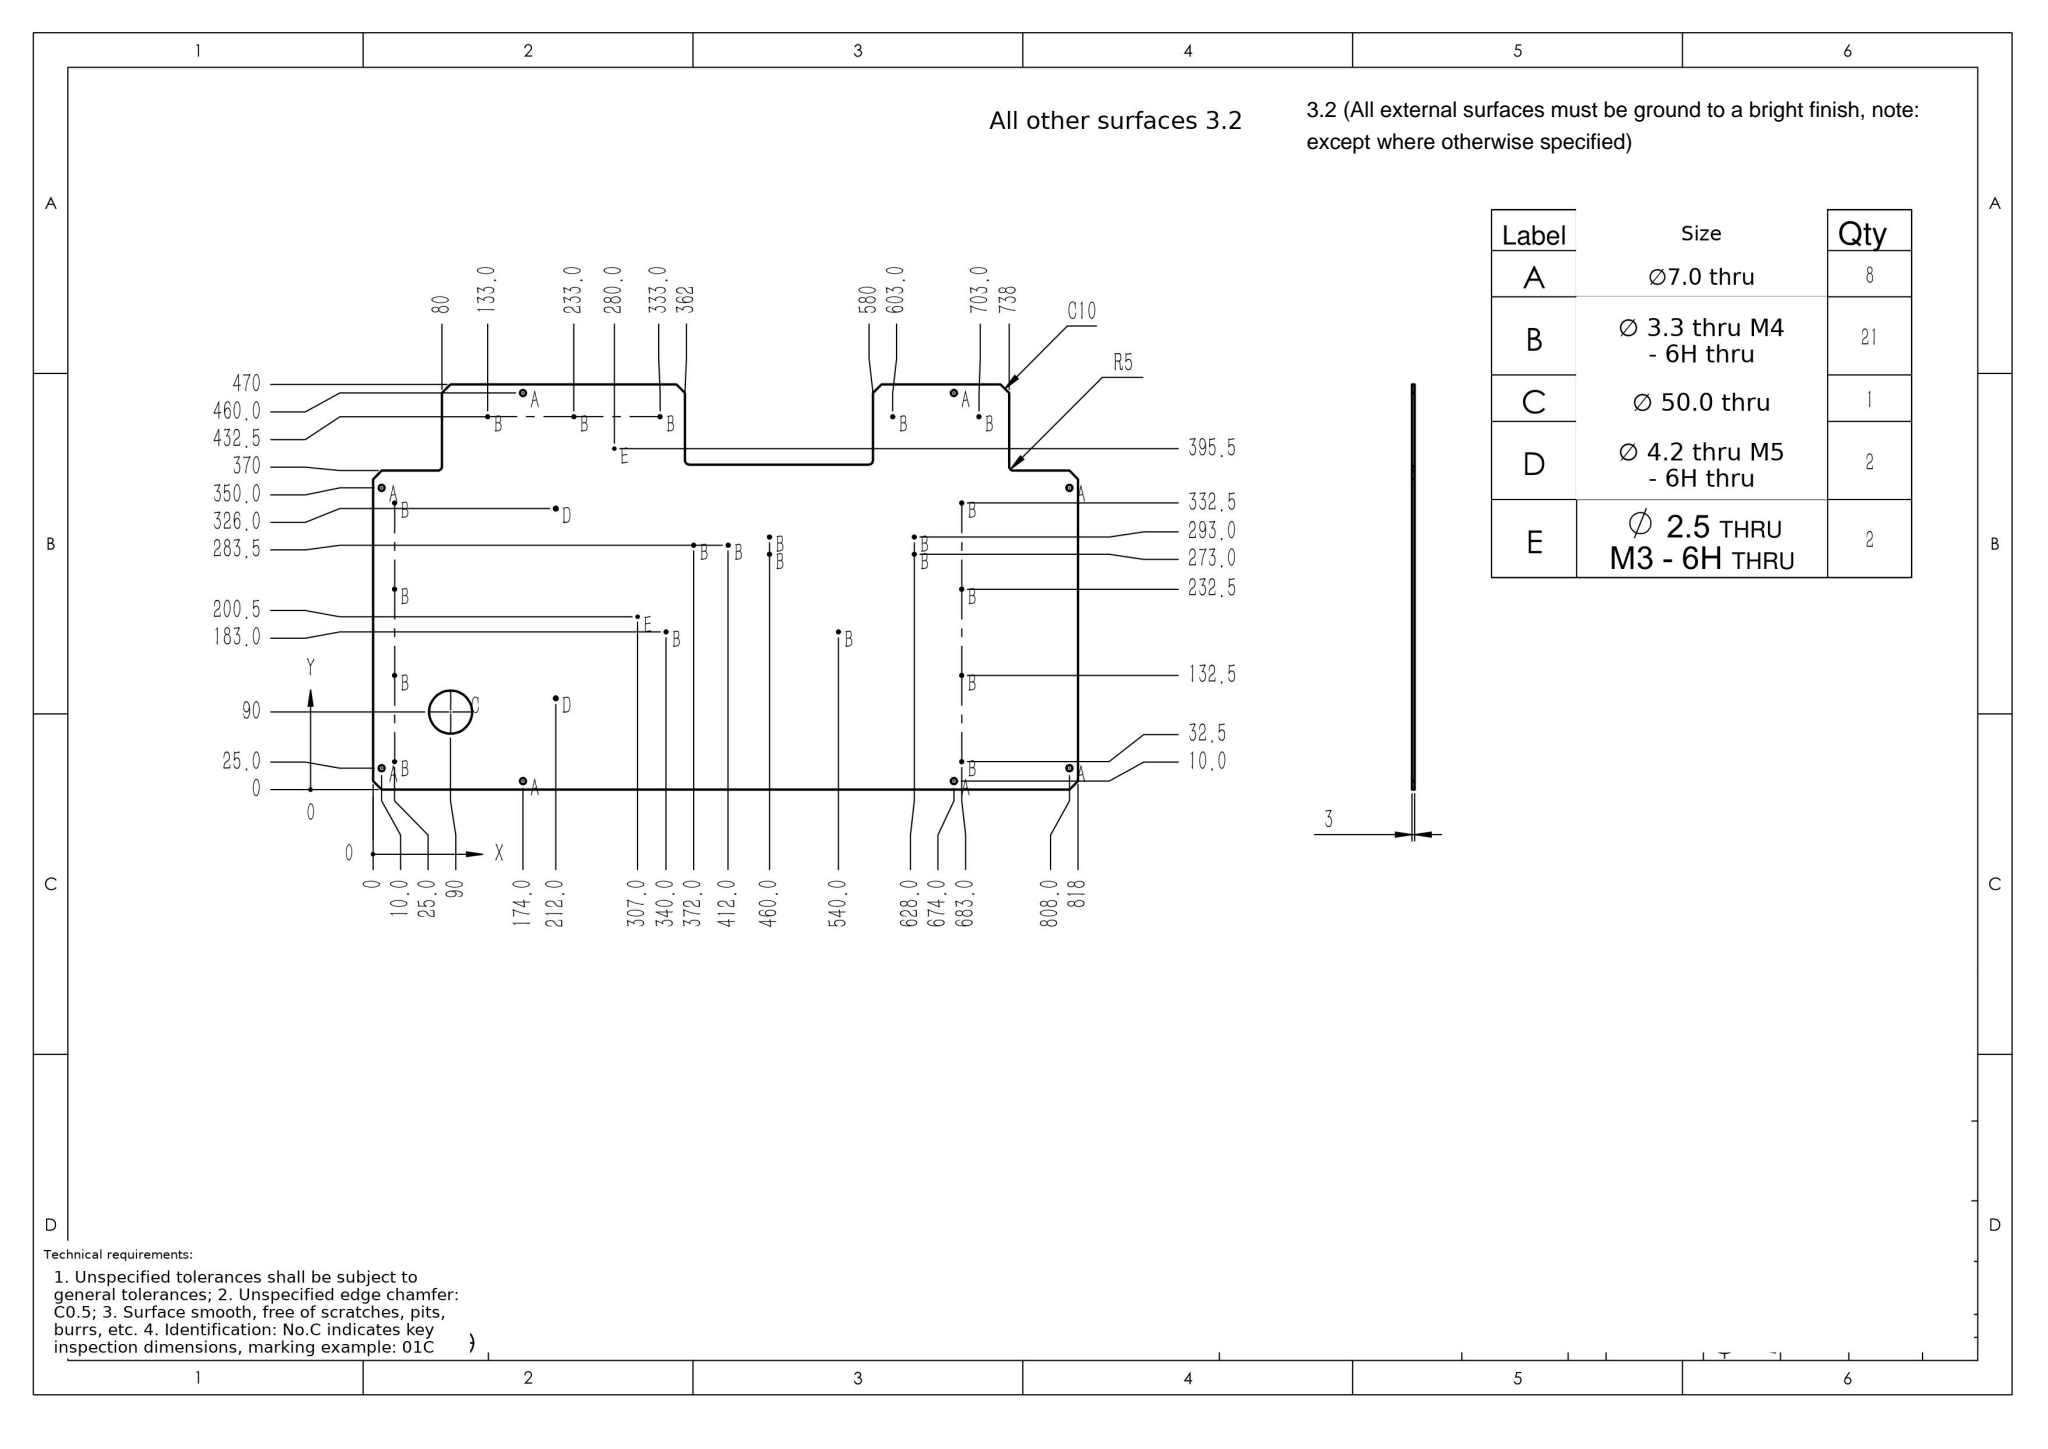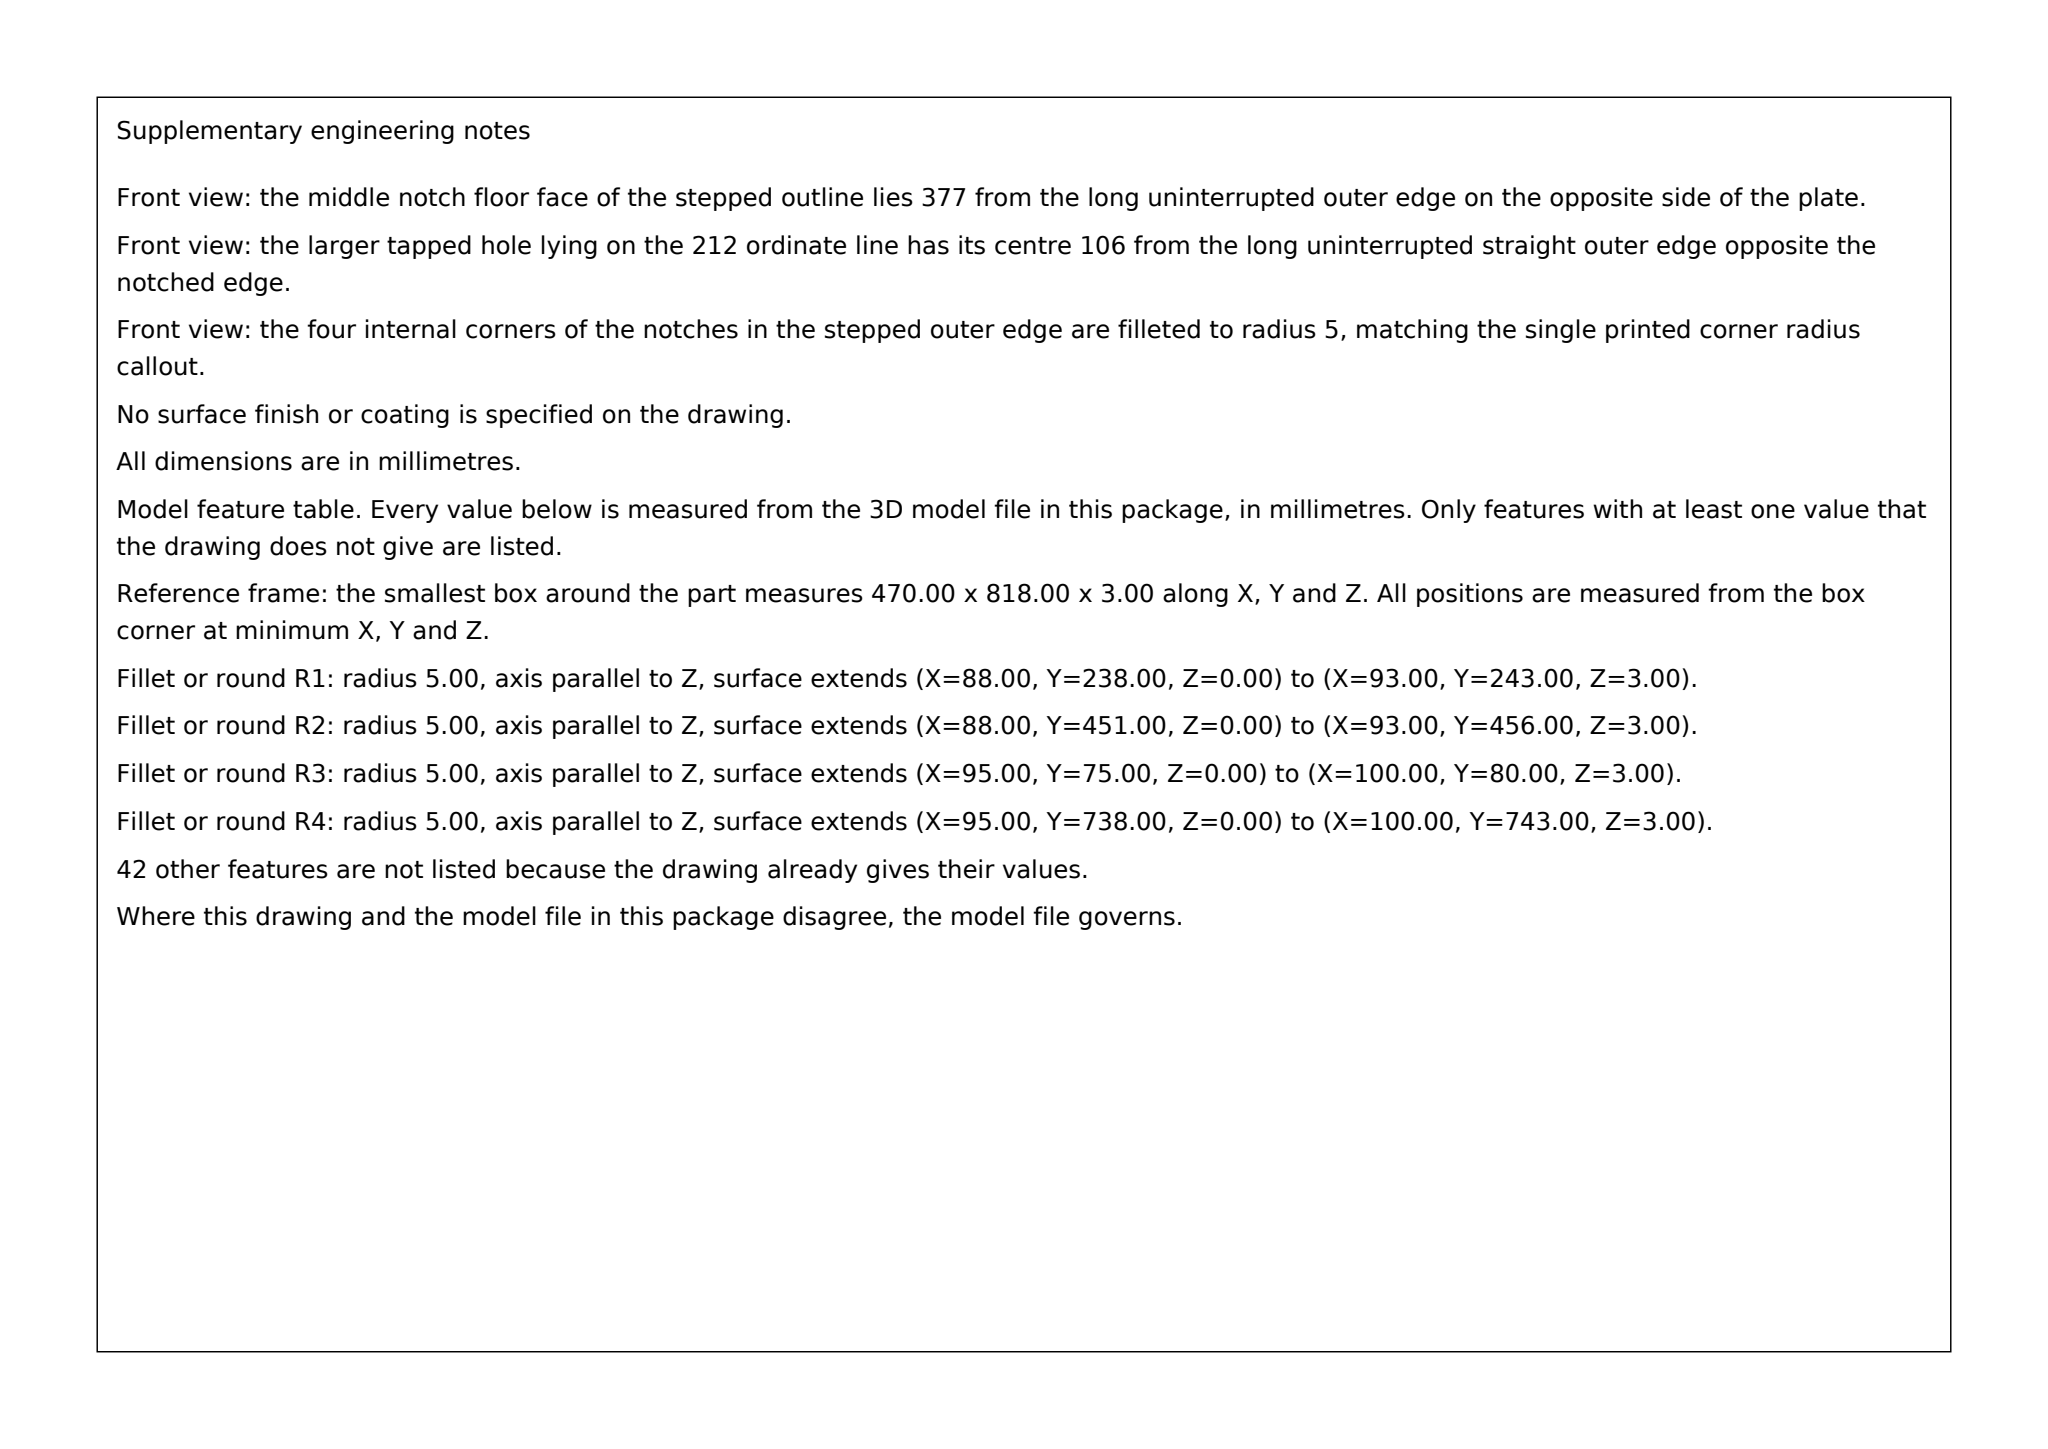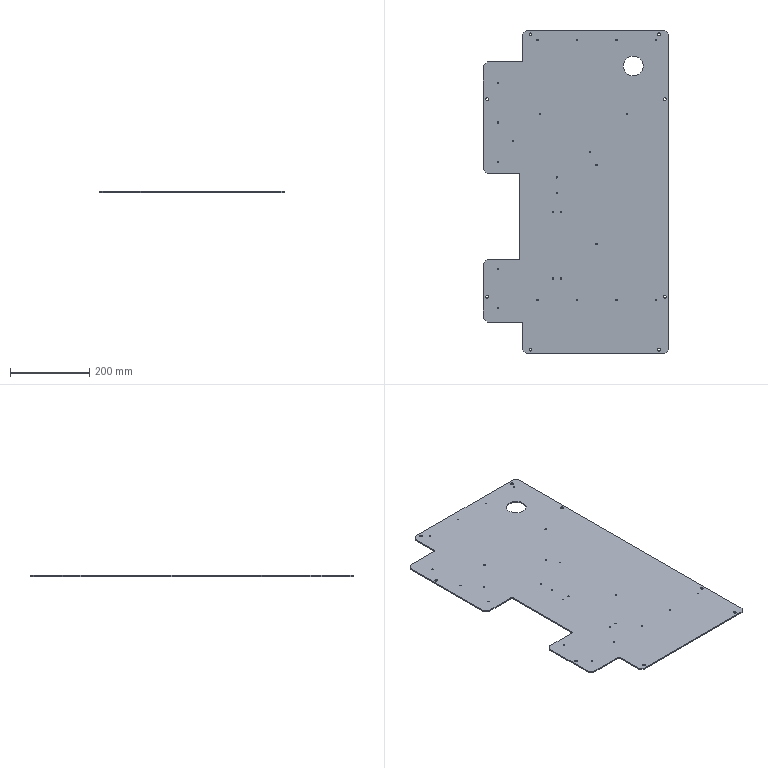Part | SolidWorks | mm | 1 solid | 94 faces | box 470 x 818 x 3 mm | volume 1035957 mm3 | cylinder 72 | plane 22 | commonest cylinder face diameters 3.3 x42 7 x16 2.5 x4 4.2 x4 10 x4 50 x2
Drawing notes:
8X C10 (45° X 10) AT ALL 8 OUTER CORNERS | from the solid: 8 inclined planes, angle_to_xyz [45,45,90], size 10x10x3, at corners (0,80),(0,228),(0,456),(0,728),(100,0),(100,808),(460,0),(460,808)
4X R5 CONCAVE CORNERS AT STEPS (R5 TYP ALL INSIDE CORNERS) | from the solid: Four concave arcs dia 10.0 (R5), axis z, at (88,243),(88,451),(95,743),(95,75), full 90 deg, thru 0-3
(11) 377 = Y TO STEP FACE, X 367 TO 575, FROM Y0 EDGE | from the solid: Plane normal x at x=93 spanning y 243-451 -> drawing Y=470-93=377, X=818-451=367 to 818-243=575
(12) 106.0 = Y TO D HOLE (M5-6H) AT X 212.0, FROM Y0 EDGE | from the solid: Hole dia 4.2 axis z at (364,606) -> drawing X=818-606=212.0, Y=470-364=106.0